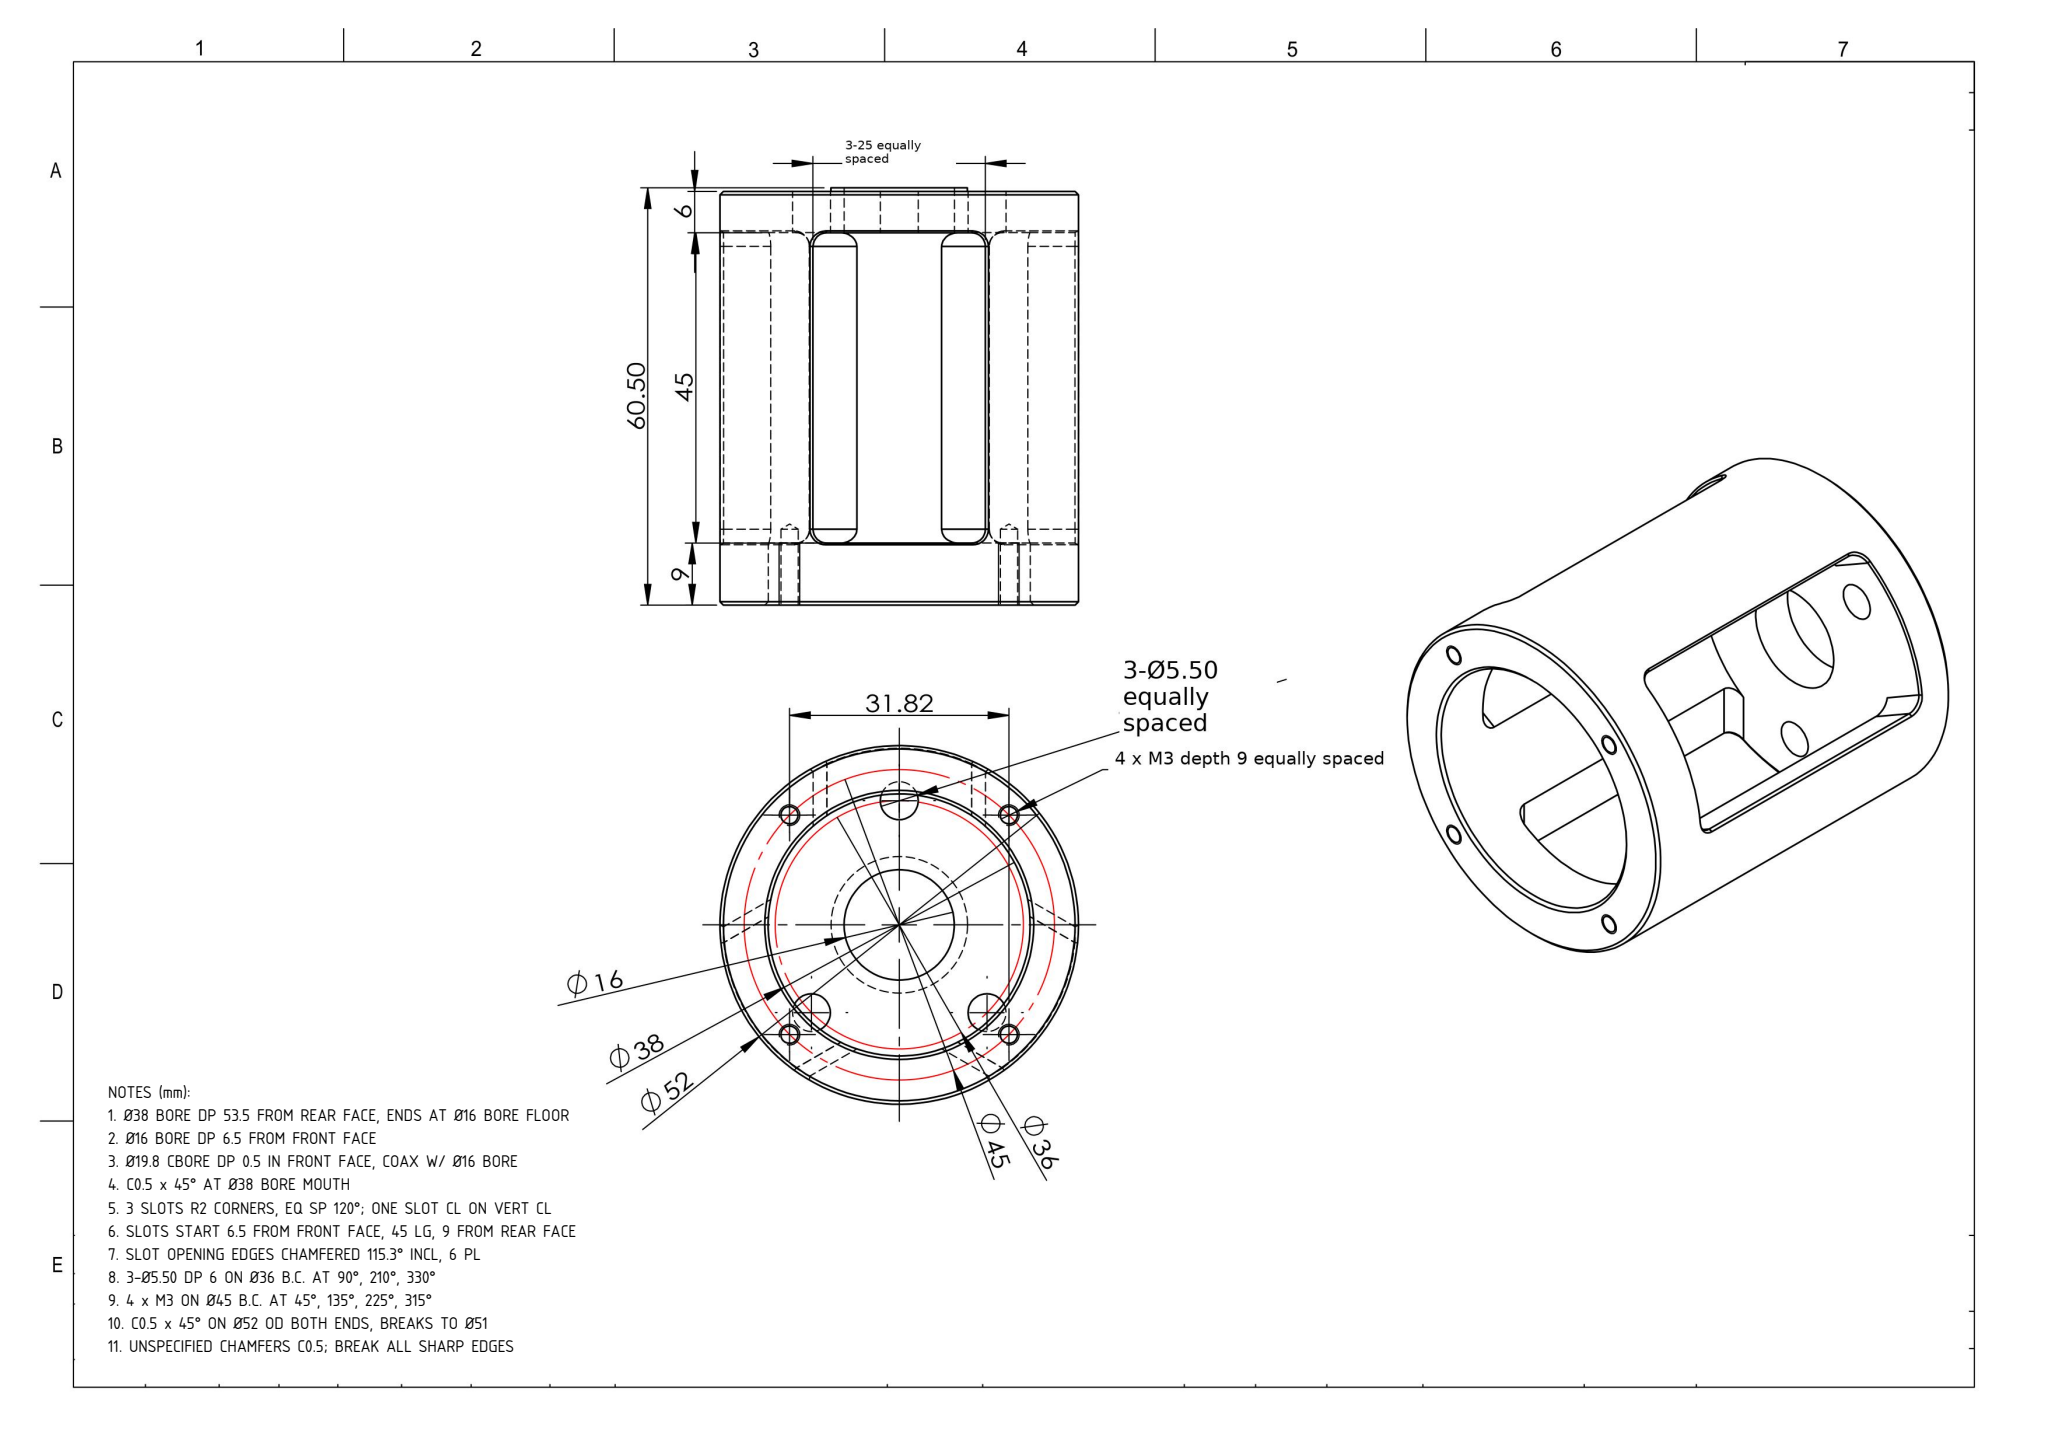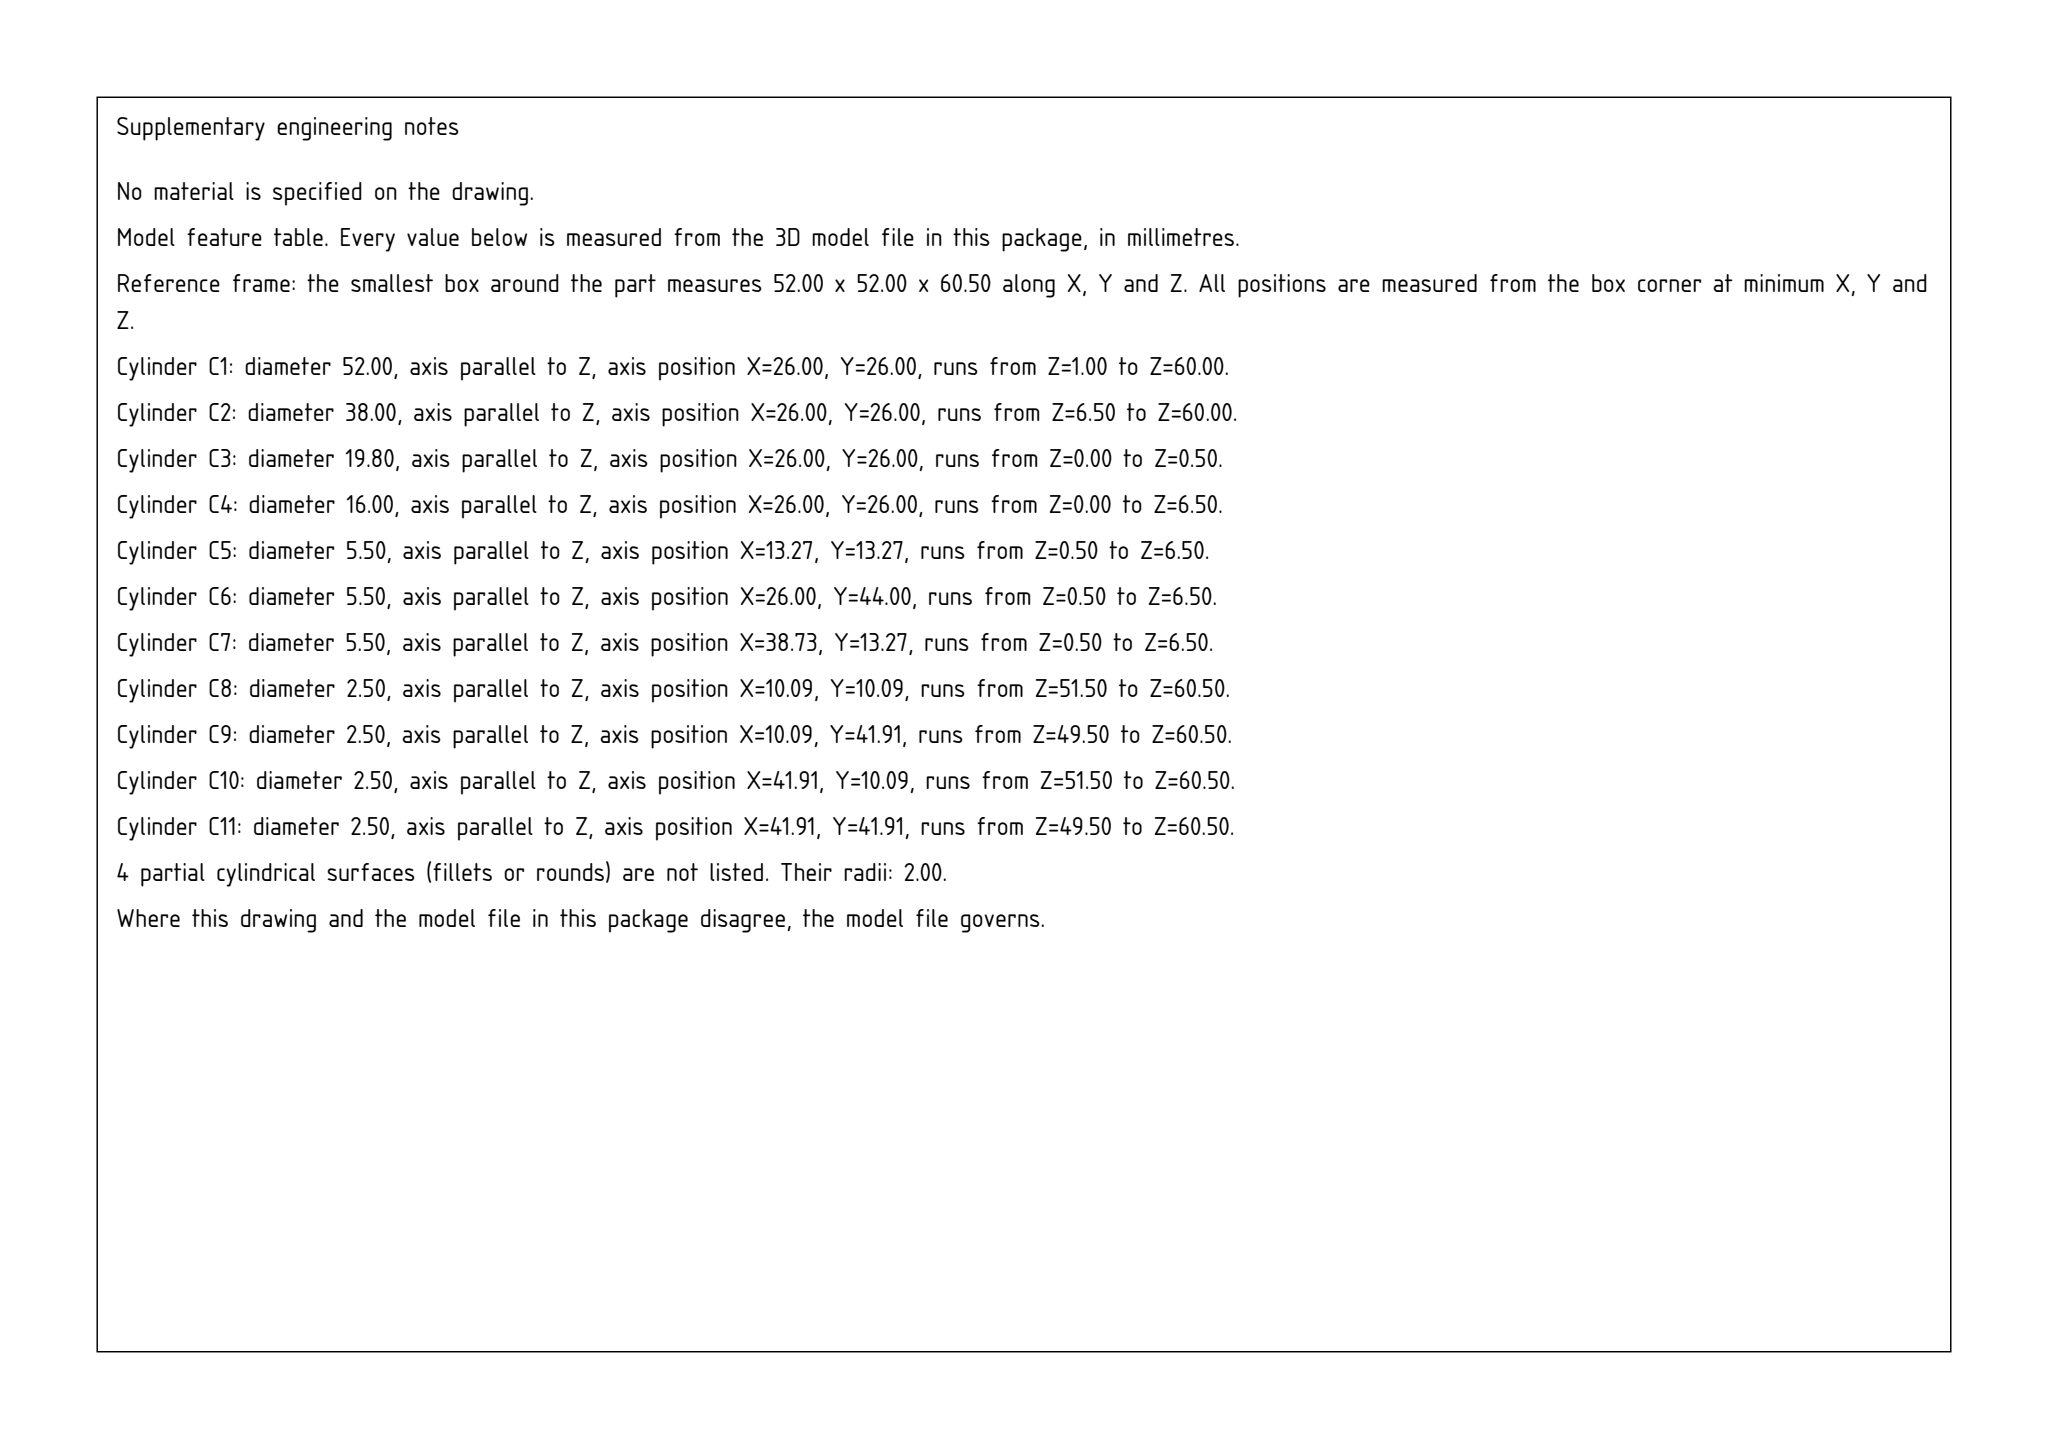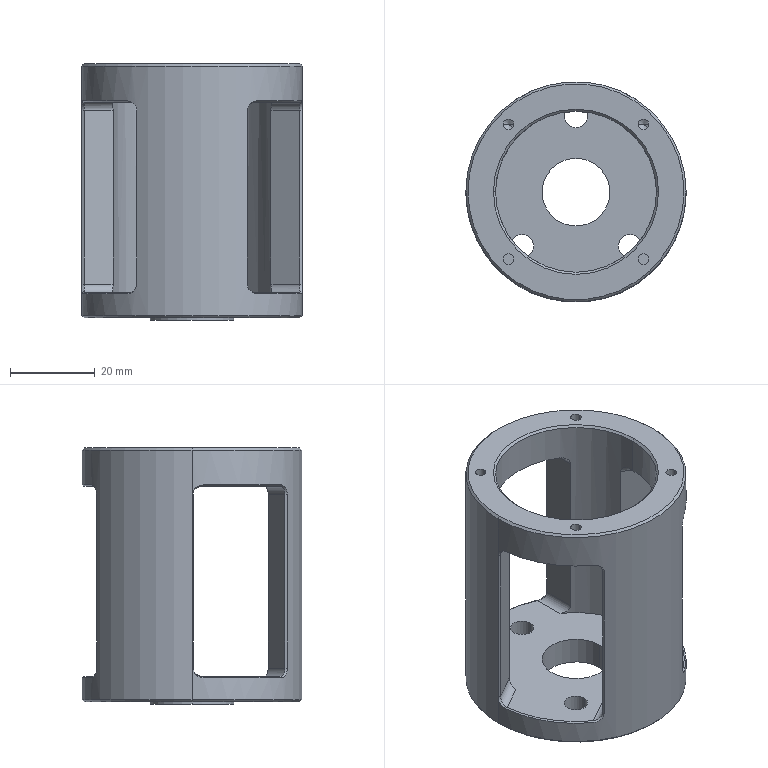Part | SolidWorks | mm | 1 solid | 81 faces | box 52 x 52 x 60.5 mm | volume 39288 mm3 | cylinder 34 | plane 19 | cone 16 | spline 12 | commonest cylinder face diameters 4 x12 2.5 x8 5.5 x6 19.8 x2 16 x2 52 x2 38 x2
Drawing notes:
Ø38 BORE DP 53.5 FROM REAR FACE, ENDS AT Ø16 BORE FLOOR | from the solid: cyl [38,z,(26.47,26.0),53.5] ends at z=6.5
Ø16 BORE DP 6.5 FROM FRONT FACE | from the solid: cyl [16,z,(26.47,26.0),6.5]; plane z=6.5
Ø19.8 CBORE DP 0.5 IN FRONT FACE, COAX W/ Ø16 BORE | from the solid: cyl [19.8,z,(26.47,26.0),0.5] from z=0; plane z=0.5
C0.5 x 45° AT Ø38 BORE MOUTH | from the solid: cone 90° incl, ref dia 38 at z=6.5 (Ø38 to Ø37)
3 SLOTS R2 CORNERS, EQ SP 120°; ONE SLOT CL ON VERT CL | from the solid: Ø4 corner cyls R2 at z=8.5 & 49.5; slot walls x=13.97/38.97, CL x=26.47
SLOTS START 6.5 FROM FRONT FACE, 45 LG, 9 FROM REAR FACE | from the solid: slot end planes z=6.5 & 51.5; bbox z=60.5
SLOT OPENING EDGES CHAMFERED 115.3° INCL, 6 PL | from the solid: cones 115.3° incl, ref dia 52, count 6 (3 slots x 2 edges)
3-Ø5.50 DP 6 ON Ø36 B.C. AT 90°, 210°, 330° | from the solid: Ø5.5 cyls len 6.0 at (26.47,44.0),(13.75,13.27),(39.2,13.27), r=18 from ctr
4 x M3 ON Ø45 B.C. AT 45°, 135°, 225°, 315° | from the solid: Ø2.5 taps at (10.56,10.09),(10.56,41.91),(42.38,10.09),(42.38,41.91), r=22.5
C0.5 x 45° ON Ø52 OD BOTH ENDS, BREAKS TO Ø51 | from the solid: cones 90° incl ref dia 52 & 51; Ø52 cyl len 59.0 vs 60.5 OAL
UNSPECIFIED CHAMFERS C0.5; BREAK ALL SHARP EDGES | from the solid: all modelled chamfers 0.5; fillet_radii empty